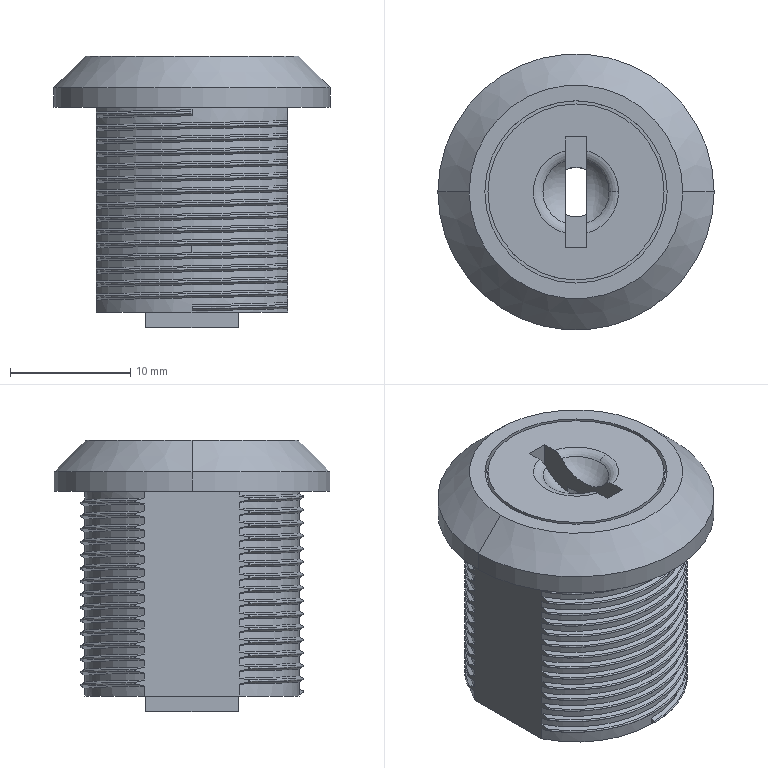Component | SolidWorks | PC-CAJ-P08-1_Chapa Guantera Duesco-1 | 1 solid | 162 faces | volume 5373 mm3 | spline 95 | cylinder 40 | plane 22 | torus 3 | cone 2 | commonest cylinder face diameters 17.78 x32 4.11 x2 22.94 x2 15.14 x2 14.62 x2 | material Plain Carbon Steel